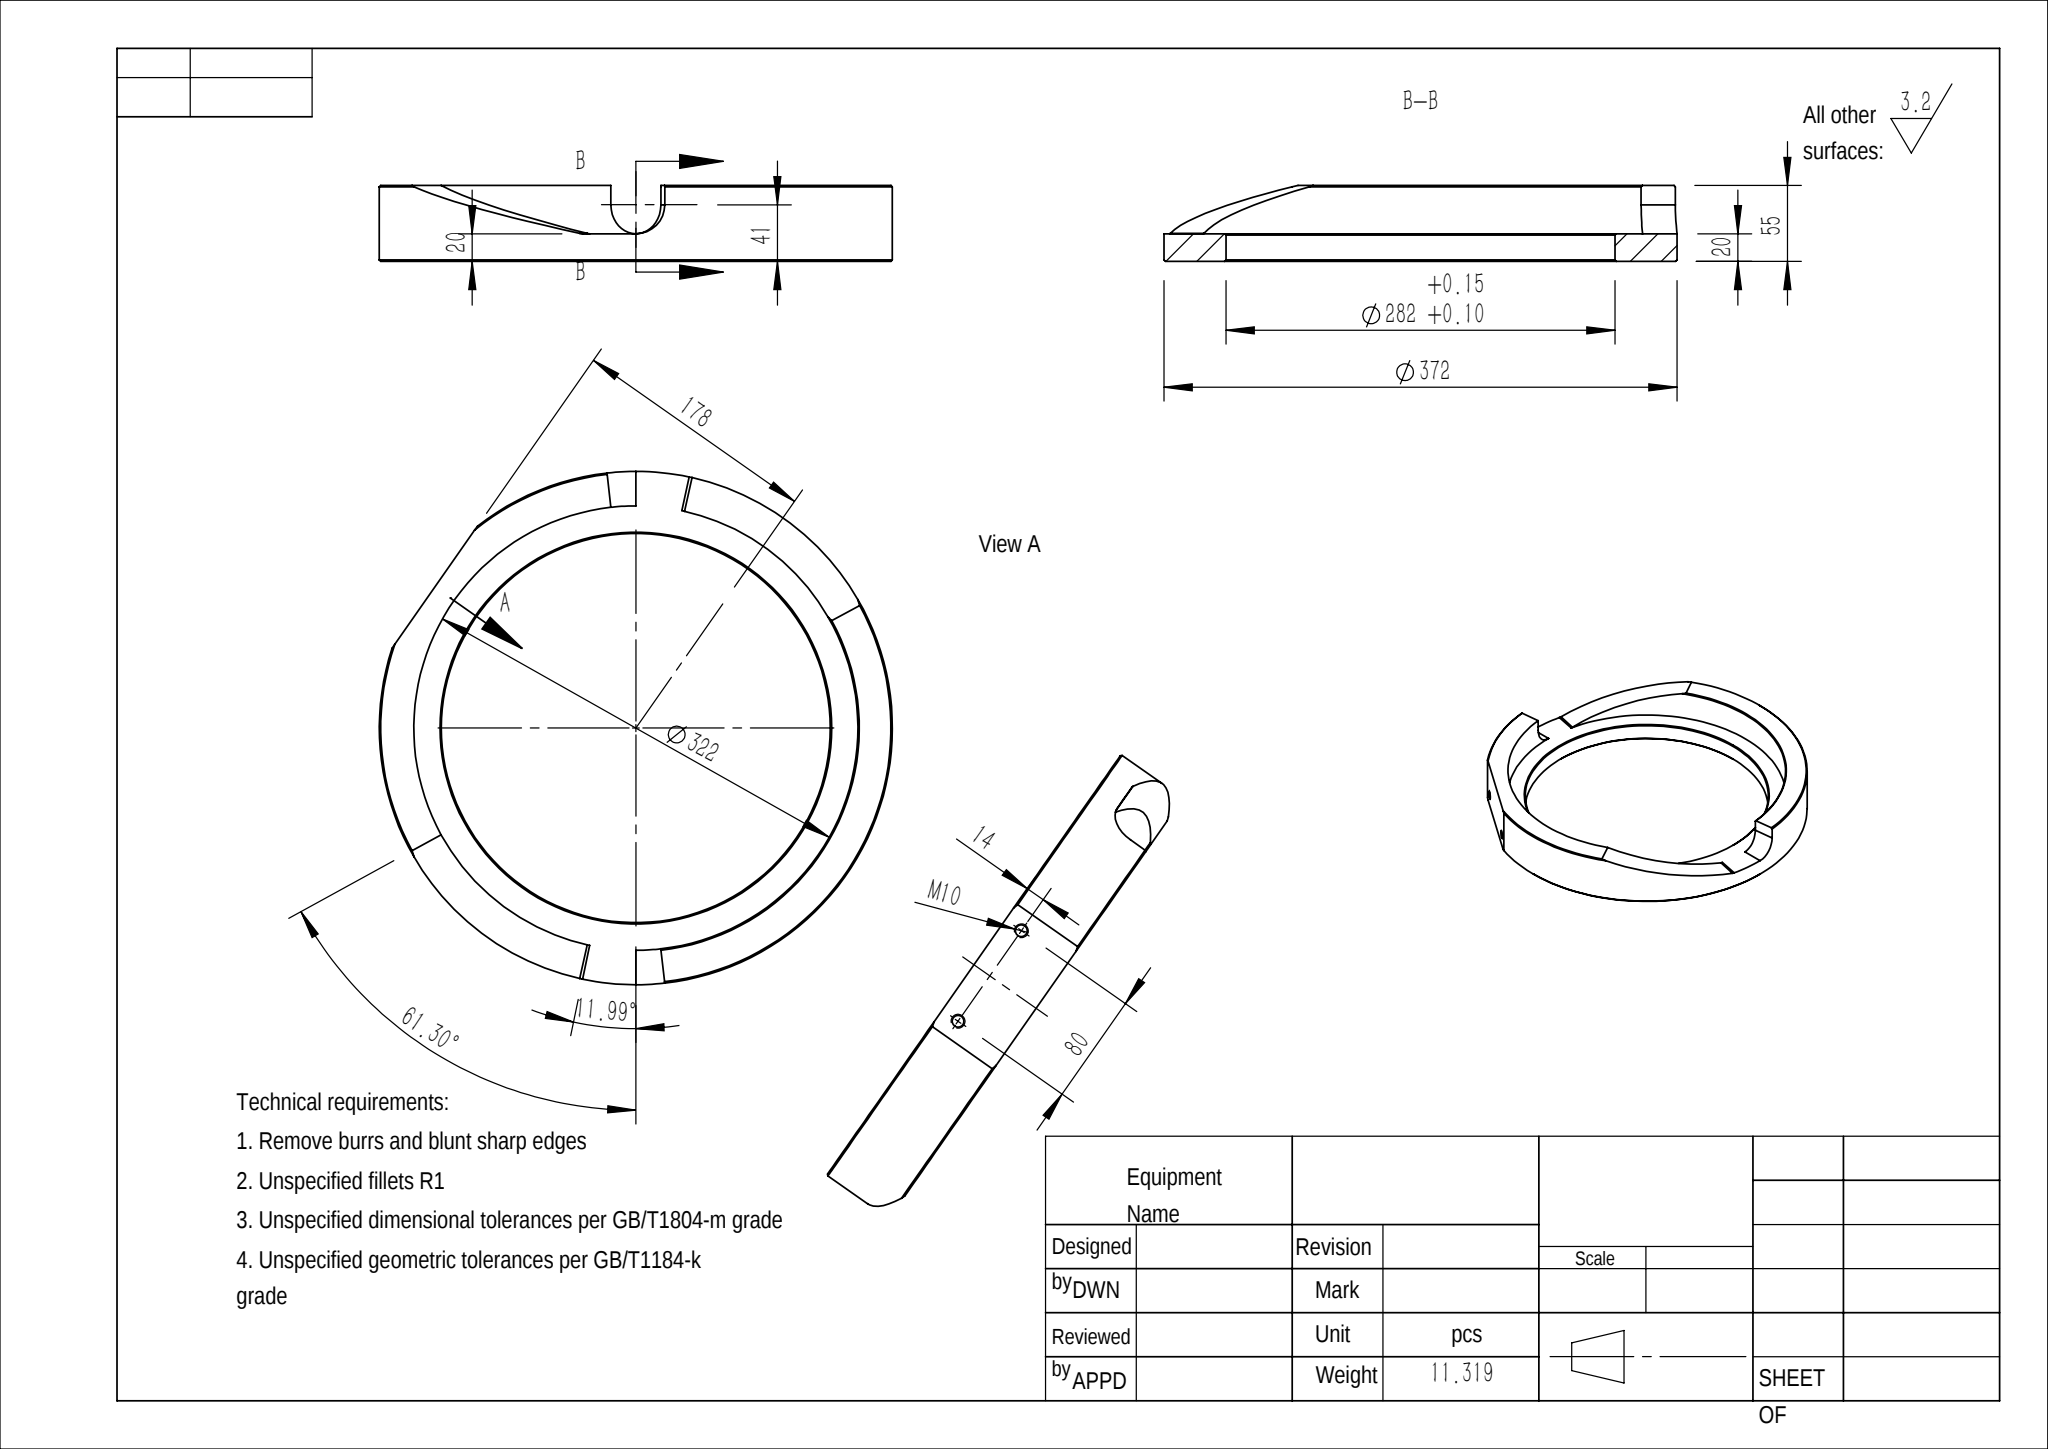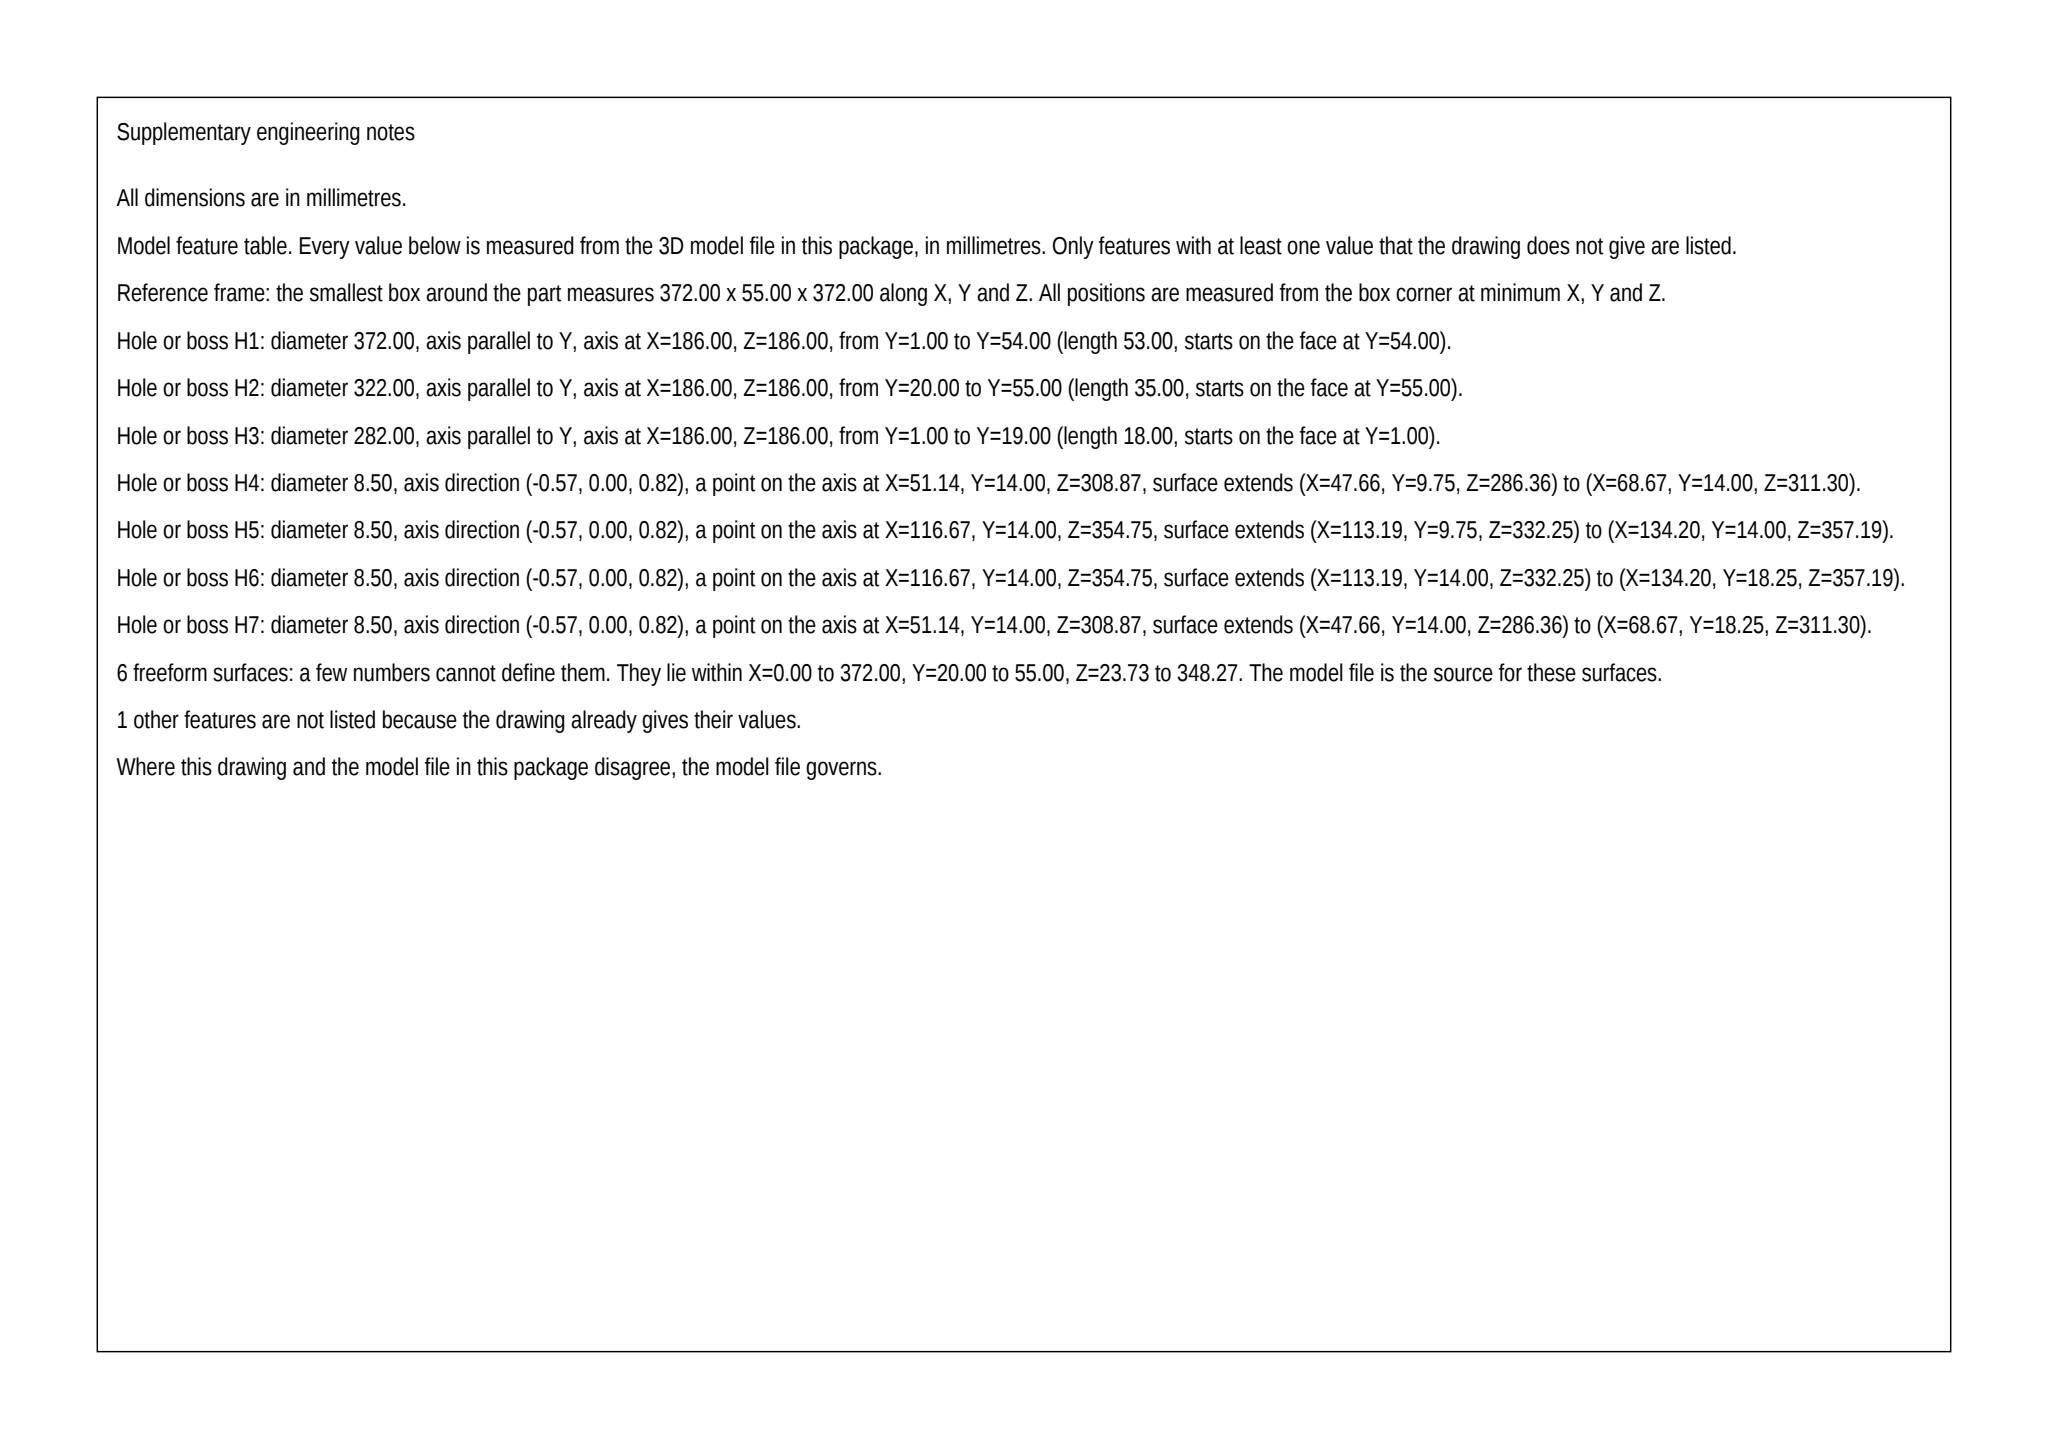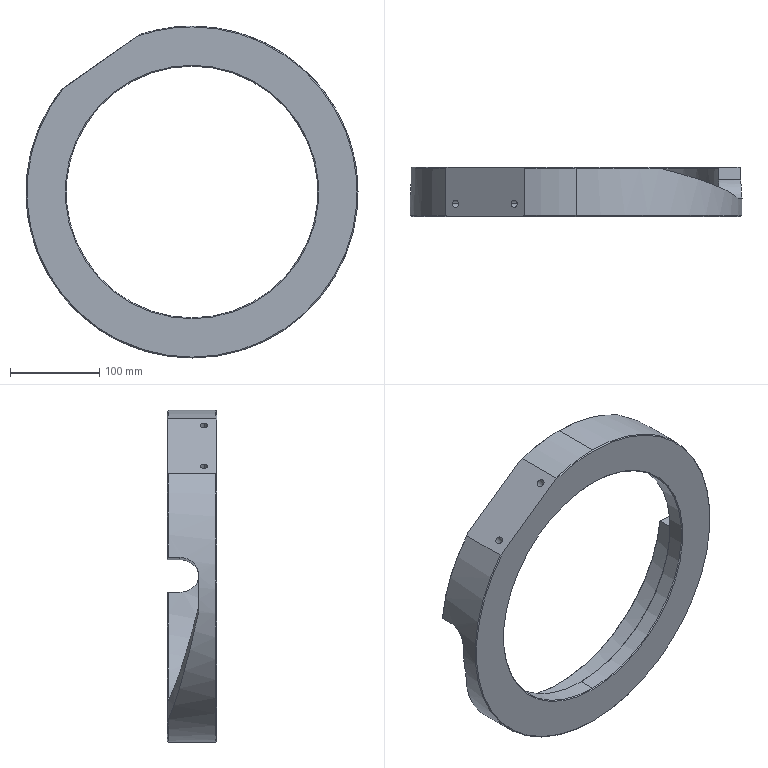Part | SolidWorks | mm | 1 solid | 41 faces | box 372 x 55 x 372 mm | volume 1616943 mm3 | cone 16 | cylinder 12 | plane 7 | spline 6 | commonest cylinder face diameters 8.5 x4 372 x3 322 x3 282 x2
Drawing notes:
VIEW A: 2X M10 THD, DRILL Ø8.5 DP 25, 118° DRILL PT | from the solid: cylinders Ø8.5 axis z, len 24.94, 2 ea at x=51.14 & 116.67, y=14; cones 118° ref dia 8.5
C1x45° ON Ø372 OD EDGE & ON Ø284 BORE EDGE | from the solid: cones 90° incl. ref dia 372/370 and 284/282 (1 mm radial drop = C1)
C1x45° ON Ø322 STEP EDGE | from the solid: cone 90° included, ref dia 322, count 1
3X NOTCH: Ø322 TO Ø372, 25 RAD DEPTH, DP 35 FROM TOP FACE | from the solid: Ø322 cyl len 34/35 vs Ø372 cyl; planes y=20 and y=55 give 35 depth; (372-322)/2=25
2X M10 DP 25 IN VIEW A: 65.53 BETWEEN CTRS, 14 FROM TOP FACE | from the solid: cylinders dia 8.5 axis z at x=51.14 and x=116.67, y=14.0, length 24.94 (2 ea) -> ctr dist 116.67-51.14=65.53
M10 HOLE PAIR CTRD ON NOTCH, 32.77 EA SIDE OF NOTCH CL | from the solid: 8.5 dia holes at x=51.14 & 116.67 symmetric about x=83.905, i.e. 32.765 each side of pair centerline